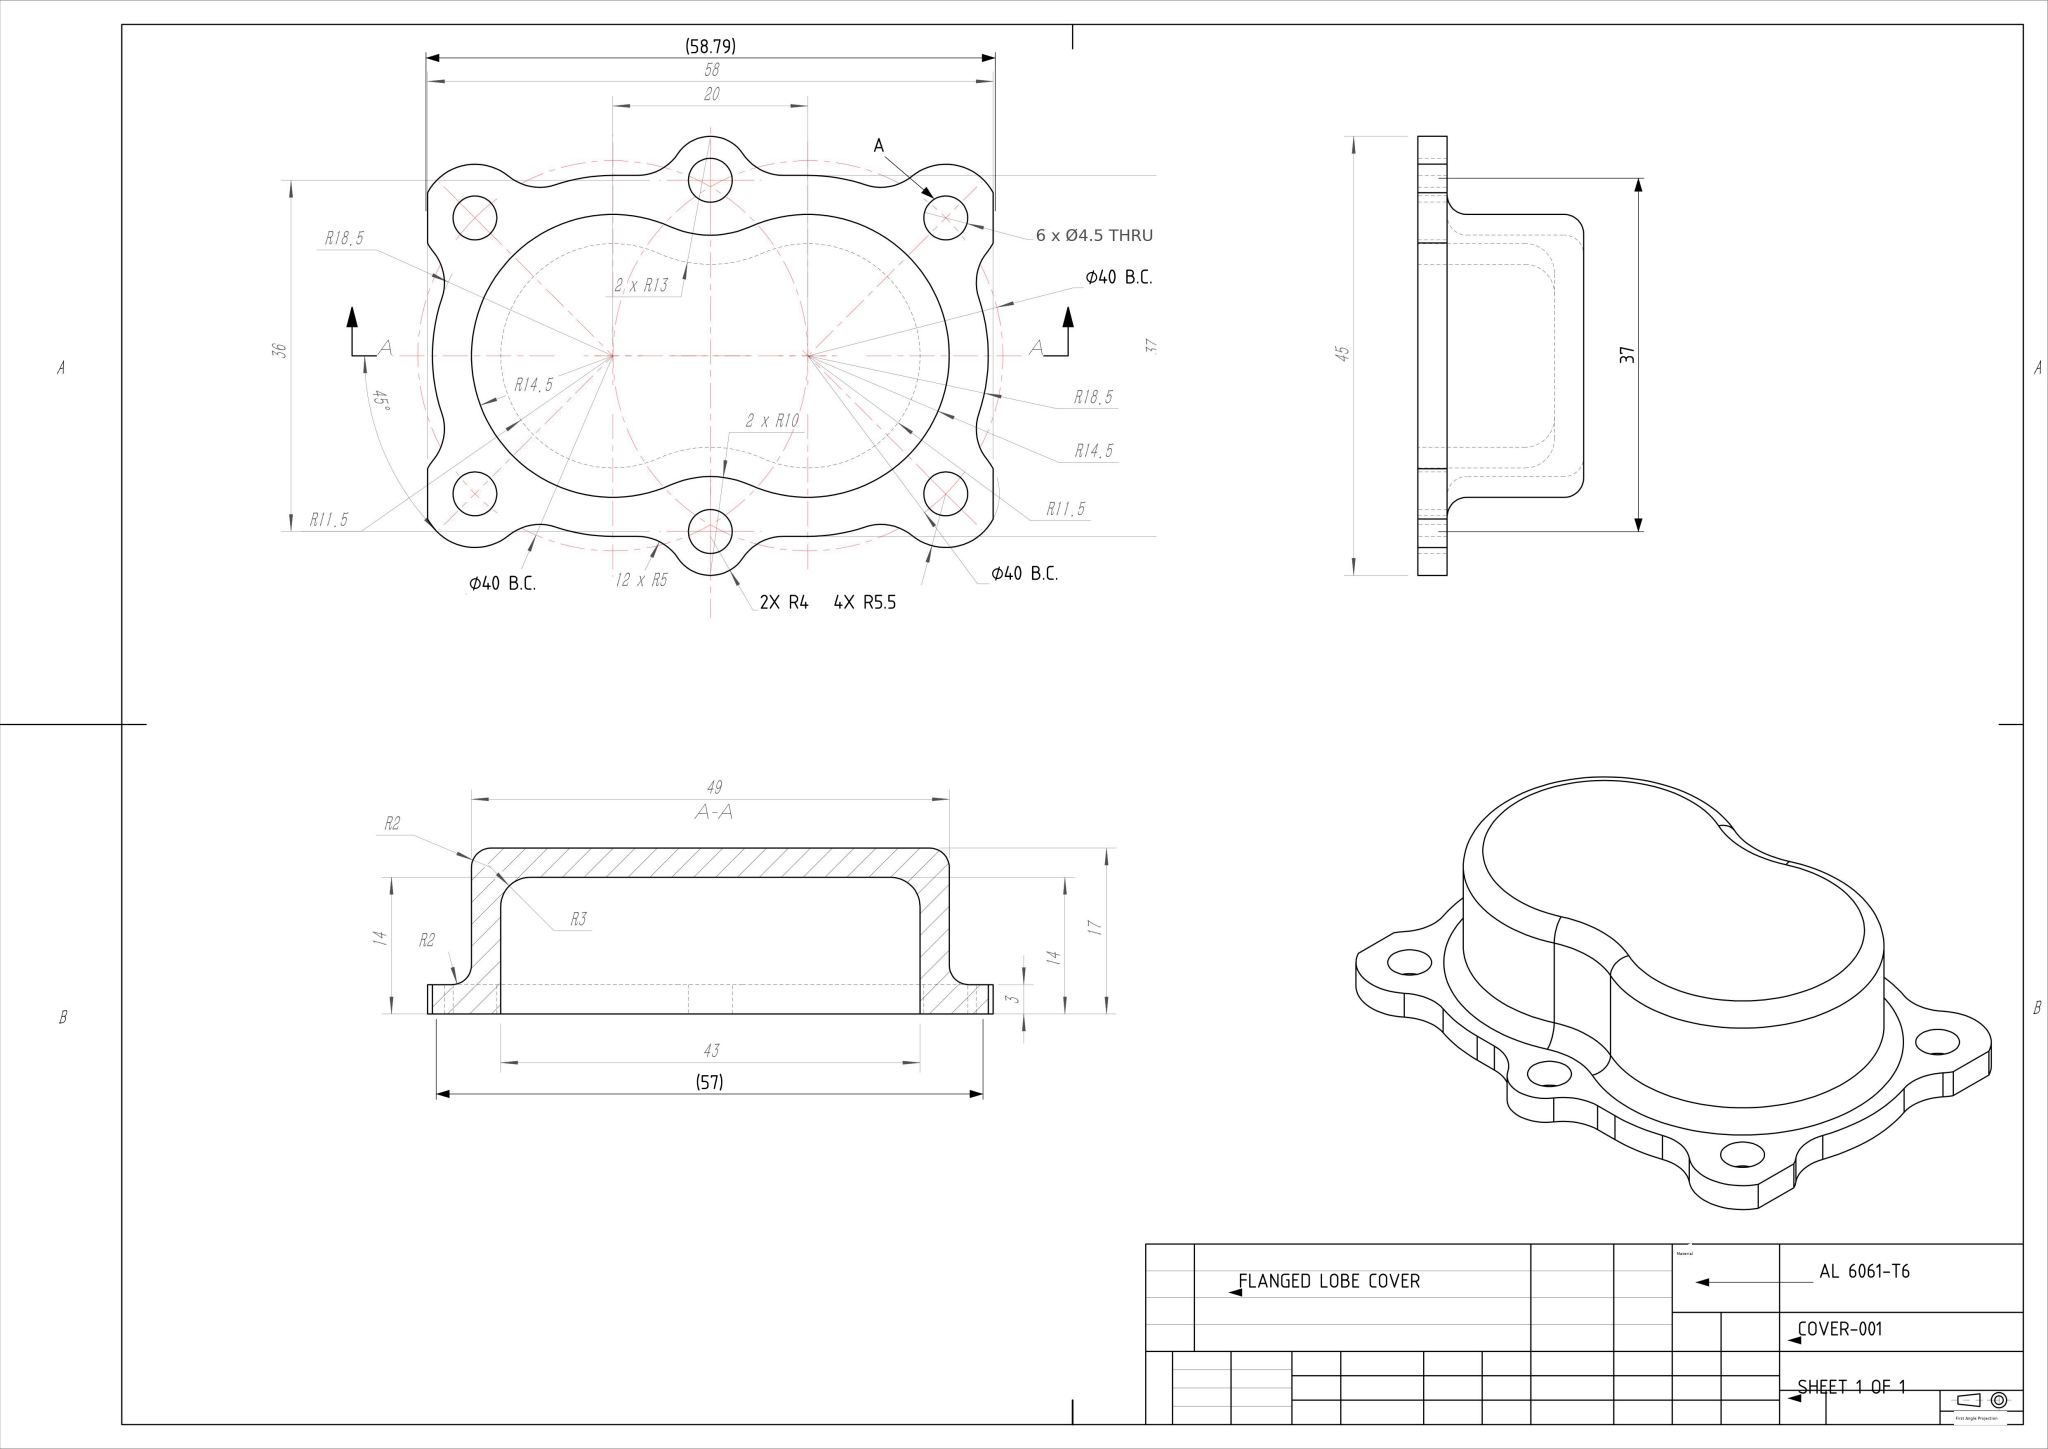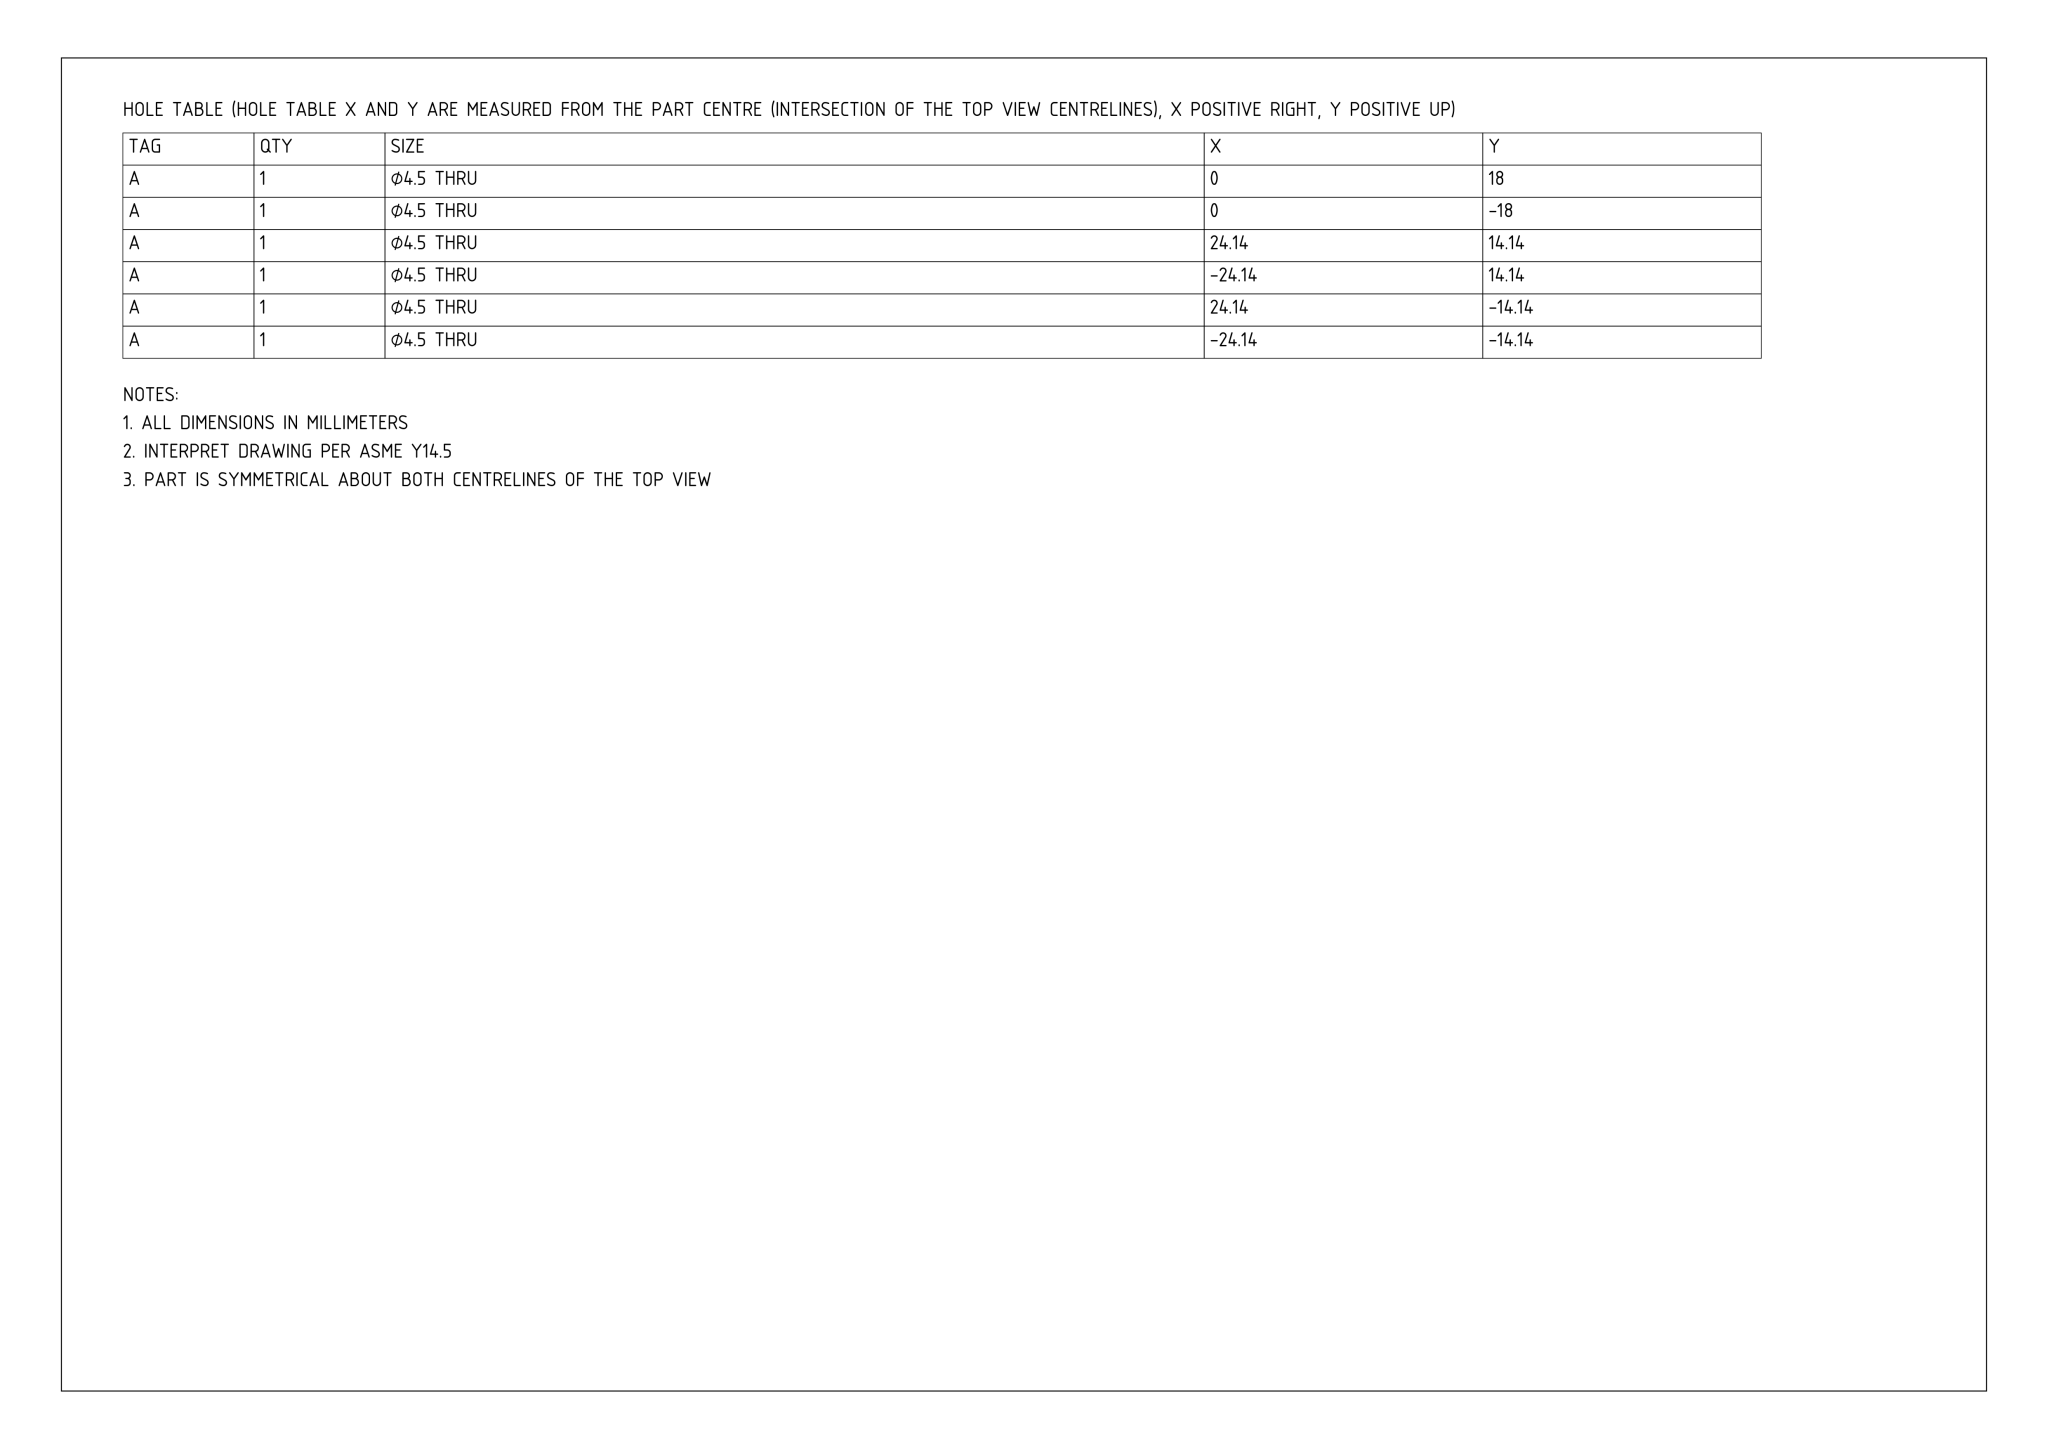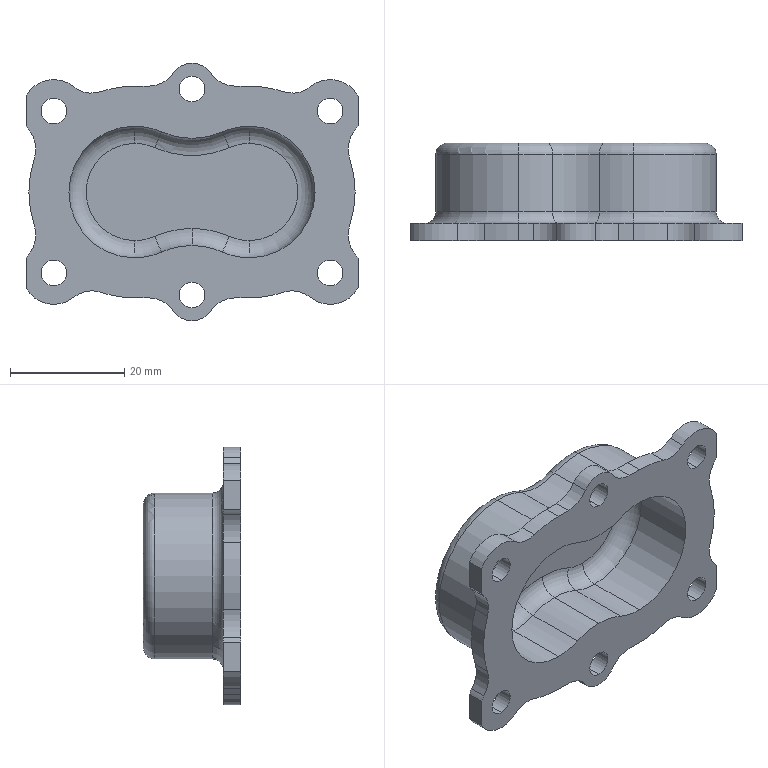Part | NX | mm | 1 solid | 102 faces | box 58 x 17 x 45 mm | volume 11527 mm3 | cylinder 63 | torus 27 | plane 12 | commonest cylinder face diameters 10 x14 4.5 x12 11 x10 23 x6 29 x6 37 x6 26 x3 20 x3